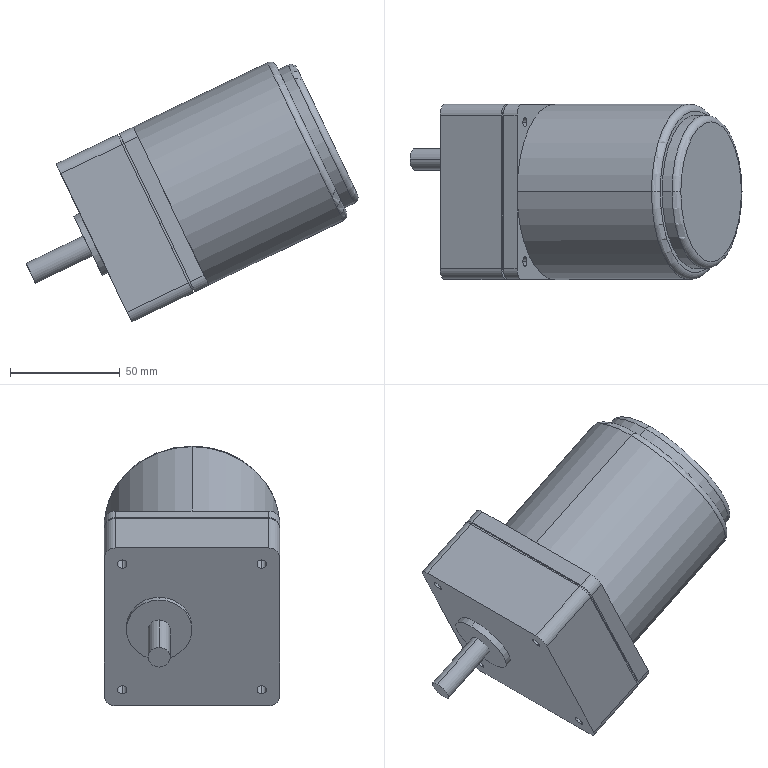Component | SolidWorks | 25WMotor-1 | 1 solid | 55 faces | box 151.57 x 80 x 118.65 mm | volume 637463 mm3 | cylinder 28 | plane 23 | torus 4 | commonest cylinder face diameters 10 x14 4.2 x8 70 x2 30 x2 80 x2
build123d program:
from build123d import *

# Parameters (mm, degrees)
SKETCH1_R           = 40
BOSS_EXTRUDE1_DEPTH = 79
SKETCH2_W           = 80
SKETCH2_H           = 80
BOSS_EXTRUDE2_DEPTH = 7
SKETCH3_W           = 78
SKETCH3_H           = 78
BOSS_EXTRUDE3_DEPTH = 1
SKETCH4_W           = 80
SKETCH4_H           = 80
BOSS_EXTRUDE4_DEPTH = 31
SKETCH5_R           = 15
BOSS_EXTRUDE5_DEPTH = 3
SKETCH6_R           = 5
BOSS_EXTRUDE6_DEPTH = 29
SKETCH7_OUTSIDE_W   = 119.576
SKETCH7_OUTSIDE_H   = 119.576
SKETCH7_OUTSIDE_R   = 35
CUT_EXTRUDE1_DEPTH  = 8
FILLET1_R           = 3
FILLET2_R           = 5
M5_TAPPED_HOLE1_D   = 4.2
CIRPATTERN1_COUNT   = 4


with BuildPart() as part:
    # Sketch1 → Boss-Extrude1 (new body)
    with BuildSketch(Plane.XY):
        Circle(SKETCH1_R)
    extrude(amount=BOSS_EXTRUDE1_DEPTH)

    # Sketch2 → Boss-Extrude2 (add)
    with BuildSketch(Plane.XY.offset(79)):
        Rectangle(SKETCH2_W, SKETCH2_H)
    extrude(amount=BOSS_EXTRUDE2_DEPTH)

    # Sketch3 → Boss-Extrude3 (add)
    with BuildSketch(Plane.XY.offset(86)):
        Rectangle(SKETCH3_W, SKETCH3_H)
    extrude(amount=BOSS_EXTRUDE3_DEPTH)

    # Sketch4 → Boss-Extrude4 (add)
    with BuildSketch(Plane.XY.offset(87)):
        Rectangle(SKETCH4_W, SKETCH4_H)
    extrude(amount=BOSS_EXTRUDE4_DEPTH)

    # Sketch5 → Boss-Extrude5 (add)
    with BuildSketch(Plane.XY.offset(118)):
        with Locations((0, 15)):
            Circle(SKETCH5_R)
    extrude(amount=BOSS_EXTRUDE5_DEPTH)

    # Sketch6 → Boss-Extrude6 (add)
    with BuildSketch(Plane.XY.offset(121)):
        with Locations(Location((0, 15, 0), (0, 0, 180))):
            Circle(SKETCH6_R)
    extrude(amount=BOSS_EXTRUDE6_DEPTH)

    # Sketch7 outside → Cut-Extrude1 (cut)
    with BuildSketch(Plane(origin=(0, 0, 0), x_dir=(-1, 0, 0), z_dir=(0, 0, -1))):
        Rectangle(SKETCH7_OUTSIDE_W, SKETCH7_OUTSIDE_H)
        Circle(SKETCH7_OUTSIDE_R, mode=Mode.SUBTRACT)
    extrude(amount=-CUT_EXTRUDE1_DEPTH, mode=Mode.SUBTRACT)

    # Fillet1
    fillet1_edges = [part.edges().sort_by_distance(p)[0] for p in [
        (-40, 0, 8),
        (35, 0, 0),
    ]]
    fillet(fillet1_edges, radius=FILLET1_R)

    # Fillet2
    fillet2_edges = [part.edges().sort_by_distance(p)[0] for p in [
        (39, -39, 86.5),
        (39, 39, 86.5),
        (-39, 39, 86.5),
        (-39, -39, 86.5),
        (40, -40, 102.5),
        (40, 40, 102.5),
        (-40, 40, 102.5),
        (-40, -40, 102.5),
        (40, -40, 82.5),
        (40, 40, 82.5),
        (-40, 40, 82.5),
        (-40, -40, 82.5),
    ]]
    fillet(fillet2_edges, radius=FILLET2_R)

    # M5 Tapped Hole1 (through all)
    with Locations(Plane(origin=(-31.82, 31.82, 118), x_dir=(1, 0, 0), z_dir=(0, 0, 1))):
        with Locations((0, 0)):
            m5_tapped_hole1 = Hole(M5_TAPPED_HOLE1_D / 2)

    # CirPattern1: M5 Tapped Hole1 ×4 about axis
    cirpattern1_axis = Axis((0, 0, 0), (0, 0, 1))
    for i in range(1, CIRPATTERN1_COUNT):
        add(m5_tapped_hole1.rotate(cirpattern1_axis, i * 360 / CIRPATTERN1_COUNT), mode=Mode.SUBTRACT)


solid = part.part

# Placed as in the assembly
solid = solid.moved(Location((92.365, 282.511, 630.092), (180, -64.419, 180)))